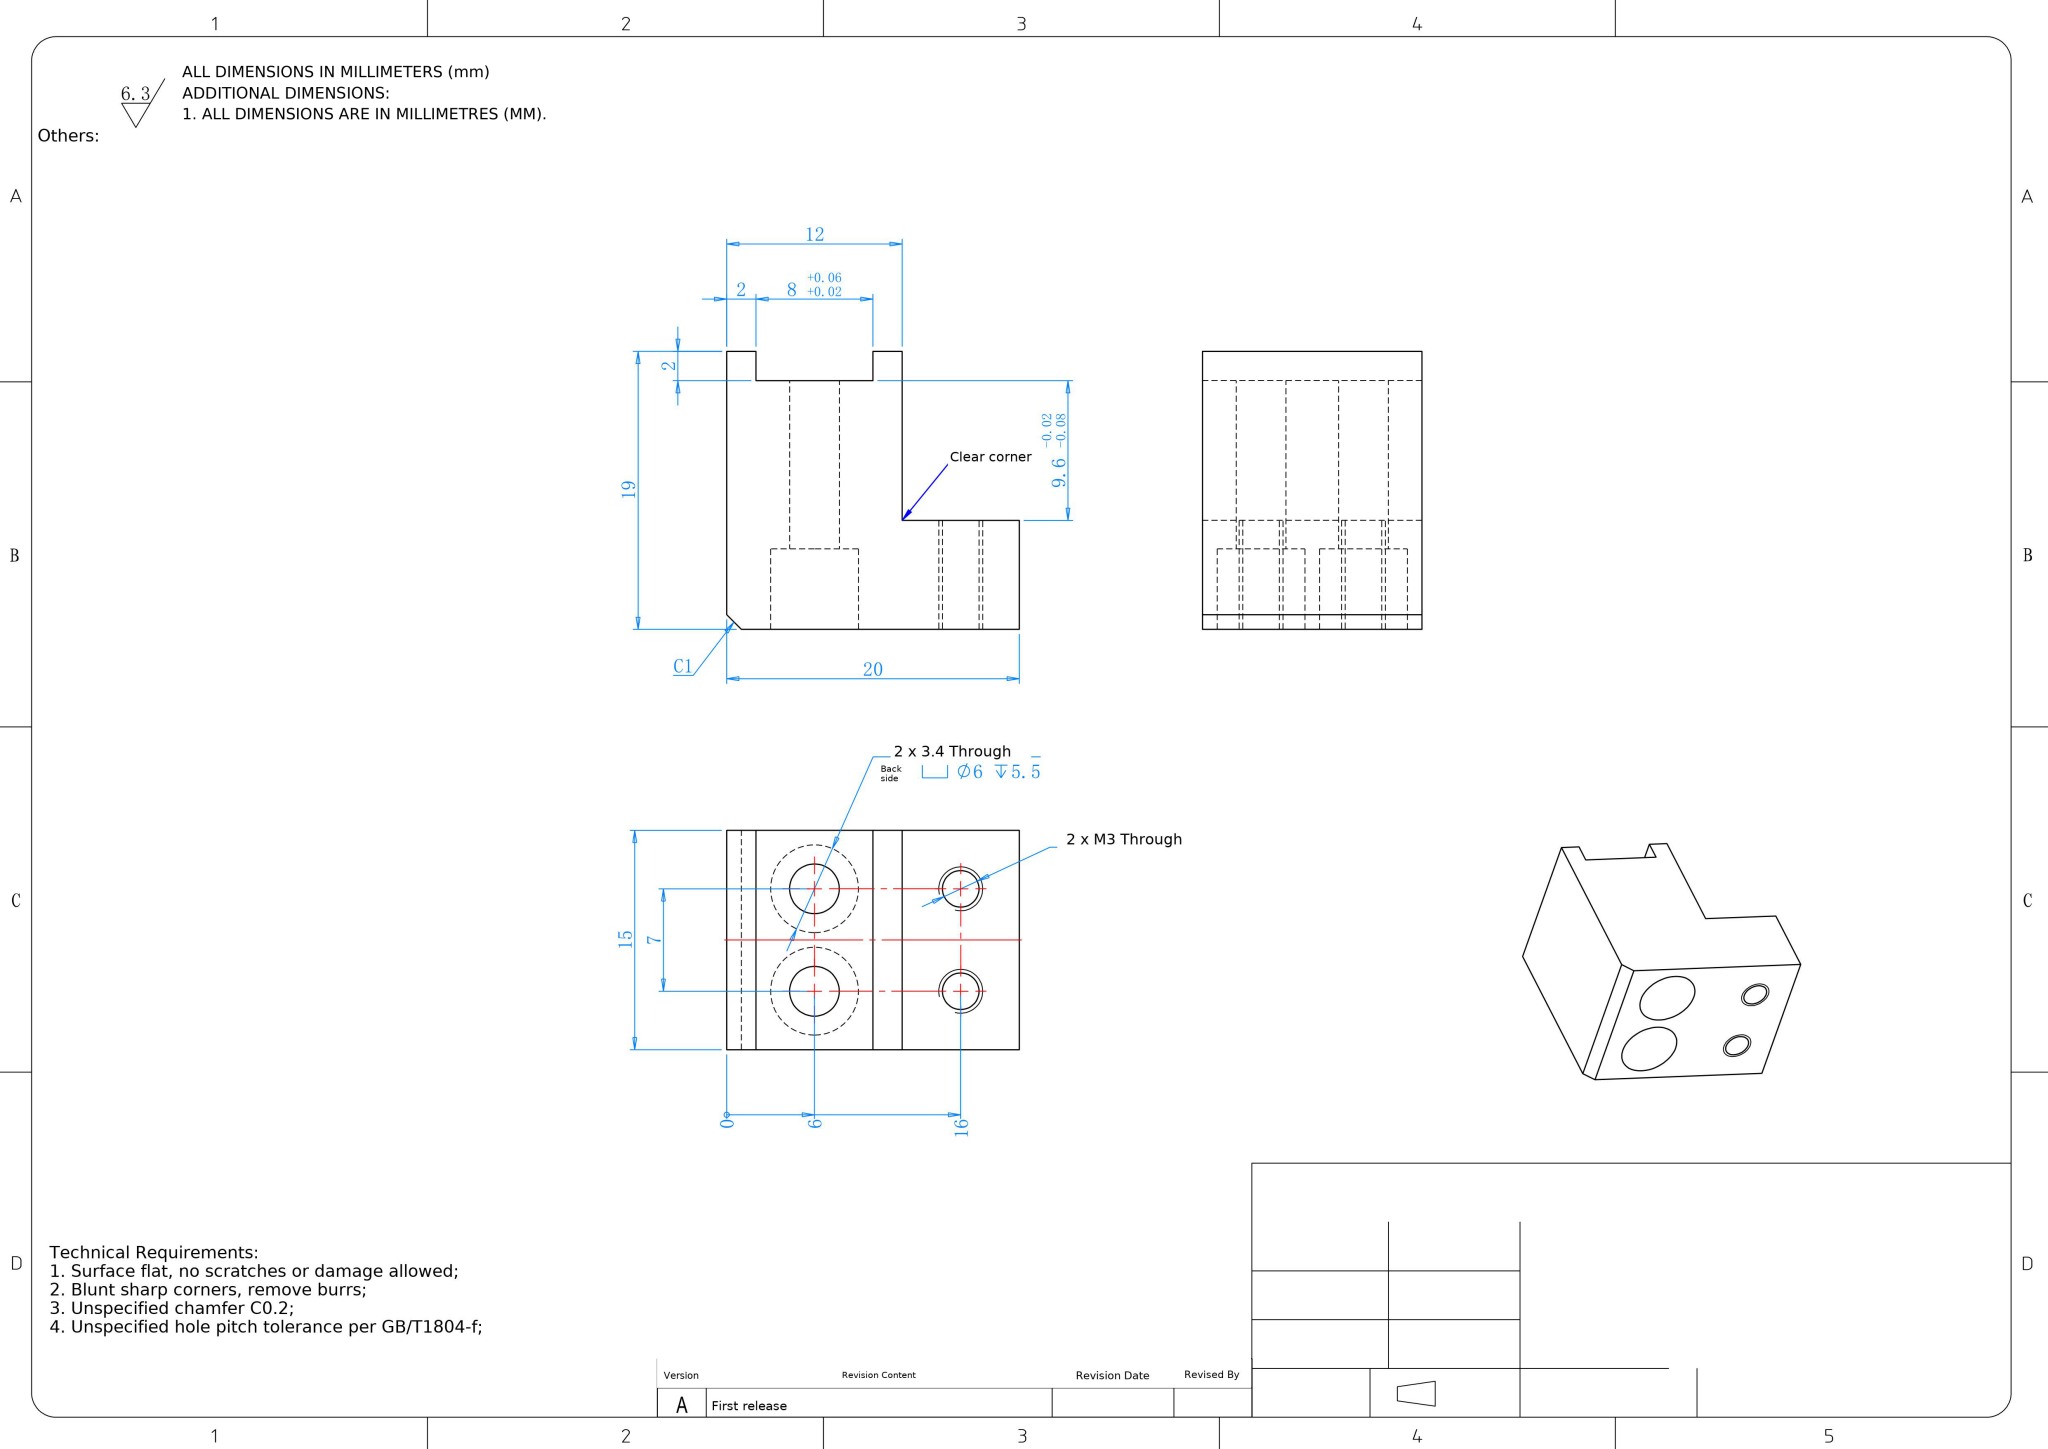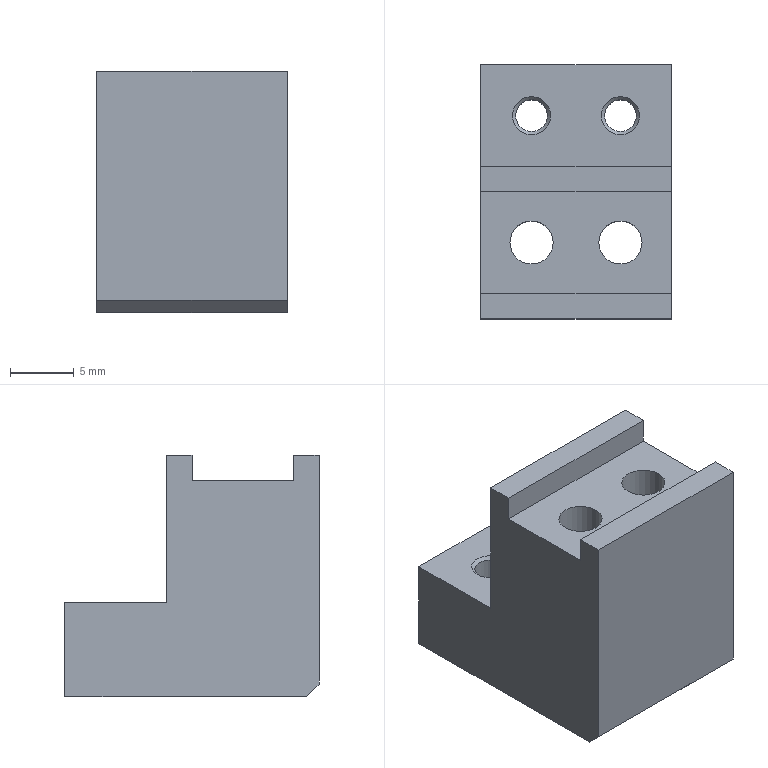Part | NX | mm | Stepped Dual-Tower Mounting Bracket | 1 solid | 25 faces | box 15 x 20 x 19 mm | volume 3467 mm3 | plane 15 | cylinder 6 | cone 4 | commonest cylinder face diameters 2.5 x2 3.4 x2 6 x2
STEP:
#1=CARTESIAN_POINT('',(0.,0.,0.));
#2=DIRECTION('',(0.,0.,1.));
#3=DIRECTION('',(1.,0.,0.));
#4=AXIS2_PLACEMENT_3D('',#1,#2,#3);
#5=(LENGTH_UNIT()NAMED_UNIT(*)SI_UNIT(.MILLI.,.METRE.));
#6=UNCERTAINTY_MEASURE_WITH_UNIT(LENGTH_MEASURE(0.00002),#5,'','');
#7=(NAMED_UNIT(*)PLANE_ANGLE_UNIT()SI_UNIT($,.RADIAN.));
#8=PLANE_ANGLE_MEASURE_WITH_UNIT(PLANE_ANGLE_MEASURE(0.01745),#7);
#9=DIMENSIONAL_EXPONENTS(0.,0.,0.,0.,0.,0.,0.);
#10=(CONVERSION_BASED_UNIT('',#8)NAMED_UNIT(#9)PLANE_ANGLE_UNIT());
#11=(NAMED_UNIT(*)SI_UNIT($,.STERADIAN.)SOLID_ANGLE_UNIT());
#12=(GEOMETRIC_REPRESENTATION_CONTEXT(3)GLOBAL_UNCERTAINTY_ASSIGNED_CONTEXT((#6))GLOBAL_UNIT_ASSIGNED_CONTEXT((#5,#10,#11))REPRESENTATION_CONTEXT('',''));
#13=SHAPE_REPRESENTATION('',(#4),#12);
#14=CARTESIAN_POINT('',(0.,-10.,19.));
#15=VERTEX_POINT('',#14);
#16=CARTESIAN_POINT('',(0.,-10.,1.));
#17=VERTEX_POINT('',#16);
#18=CARTESIAN_POINT('',(0.,-10.,19.));
#19=DIRECTION('',(0.,0.,-1.));
#20=VECTOR('',#19,1.);
#21=LINE('',#18,#20);
#22=EDGE_CURVE('',#15,#17,#21,.T.);
#23=ORIENTED_EDGE('',*,*,#22,.T.);
#24=CARTESIAN_POINT('',(15.,-10.,1.));
#25=VERTEX_POINT('',#24);
#26=CARTESIAN_POINT('',(15.,-10.,1.));
#27=DIRECTION('',(-1.,0.,0.));
#28=VECTOR('',#27,1.);
#29=LINE('',#26,#28);
#30=EDGE_CURVE('',#25,#17,#29,.T.);
#31=ORIENTED_EDGE('',*,*,#30,.F.);
#32=CARTESIAN_POINT('',(15.,-10.,19.));
#33=VERTEX_POINT('',#32);
#34=CARTESIAN_POINT('',(15.,-10.,19.));
#35=DIRECTION('',(0.,0.,-1.));
#36=VECTOR('',#35,1.);
#37=LINE('',#34,#36);
#38=EDGE_CURVE('',#33,#25,#37,.T.);
#39=ORIENTED_EDGE('',*,*,#38,.F.);
#40=CARTESIAN_POINT('',(15.,-10.,19.));
#41=DIRECTION('',(-1.,0.,0.));
#42=VECTOR('',#41,1.);
#43=LINE('',#40,#42);
#44=EDGE_CURVE('',#33,#15,#43,.T.);
#45=ORIENTED_EDGE('',*,*,#44,.T.);
#46=EDGE_LOOP('',(#23,#31,#39,#45));
#47=FACE_OUTER_BOUND('',#46,.T.);
#48=CARTESIAN_POINT('',(15.,-10.,19.));
#49=DIRECTION('',(0.,1.,0.));
#50=DIRECTION('',(0.,0.,1.));
#51=AXIS2_PLACEMENT_3D('',#48,#49,#50);
#52=PLANE('',#51);
#53=ADVANCED_FACE('',(#47),#52,.F.);
#54=CARTESIAN_POINT('',(0.,-9.,-0.));
#55=VERTEX_POINT('',#54);
#56=CARTESIAN_POINT('',(0.,-10.,1.));
#57=DIRECTION('',(0.,0.7071,-0.7071));
#58=VECTOR('',#57,1.);
#59=LINE('',#56,#58);
#60=EDGE_CURVE('',#17,#55,#59,.T.);
#61=ORIENTED_EDGE('',*,*,#60,.T.);
#62=CARTESIAN_POINT('',(15.,-9.,-0.));
#63=VERTEX_POINT('',#62);
#64=CARTESIAN_POINT('',(15.,-9.,-0.));
#65=DIRECTION('',(-1.,0.,0.));
#66=VECTOR('',#65,1.);
#67=LINE('',#64,#66);
#68=EDGE_CURVE('',#63,#55,#67,.T.);
#69=ORIENTED_EDGE('',*,*,#68,.F.);
#70=CARTESIAN_POINT('',(15.,-10.,1.));
#71=DIRECTION('',(0.,0.7071,-0.7071));
#72=VECTOR('',#71,1.);
#73=LINE('',#70,#72);
#74=EDGE_CURVE('',#25,#63,#73,.T.);
#75=ORIENTED_EDGE('',*,*,#74,.F.);
#76=ORIENTED_EDGE('',*,*,#30,.T.);
#77=EDGE_LOOP('',(#61,#69,#75,#76));
#78=FACE_OUTER_BOUND('',#77,.T.);
#79=CARTESIAN_POINT('',(15.,-10.,1.));
#80=DIRECTION('',(0.,0.7071,0.7071));
#81=DIRECTION('',(0.,-0.7071,0.7071));
#82=AXIS2_PLACEMENT_3D('',#79,#80,#81);
#83=PLANE('',#82);
#84=ADVANCED_FACE('',(#78),#83,.F.);
#85=CARTESIAN_POINT('',(7.,-4.,0.));
#86=VERTEX_POINT('',#85);
#87=CARTESIAN_POINT('',(4.,-4.,0.));
#88=DIRECTION('',(0.,0.,1.));
#89=DIRECTION('',(1.,0.,0.));
#90=AXIS2_PLACEMENT_3D('',#87,#88,#89);
#91=CIRCLE('',#90,3.);
#92=EDGE_CURVE('',#86,#86,#91,.T.);
#93=ORIENTED_EDGE('',*,*,#92,.T.);
#94=EDGE_LOOP('',(#93));
#95=FACE_BOUND('',#94,.T.);
#96=CARTESIAN_POINT('',(14.,-4.,0.));
#97=VERTEX_POINT('',#96);
#98=CARTESIAN_POINT('',(11.,-4.,0.));
#99=DIRECTION('',(0.,0.,1.));
#100=DIRECTION('',(1.,0.,0.));
#101=AXIS2_PLACEMENT_3D('',#98,#99,#100);
#102=CIRCLE('',#101,3.);
#103=EDGE_CURVE('',#97,#97,#102,.T.);
#104=ORIENTED_EDGE('',*,*,#103,.T.);
#105=EDGE_LOOP('',(#104));
#106=FACE_BOUND('',#105,.T.);
#107=CARTESIAN_POINT('',(5.5,6.,0.));
#108=VERTEX_POINT('',#107);
#109=CARTESIAN_POINT('',(4.,6.,0.));
#110=DIRECTION('',(0.,0.,1.));
#111=DIRECTION('',(1.,0.,0.));
#112=AXIS2_PLACEMENT_3D('',#109,#110,#111);
#113=CIRCLE('',#112,1.5);
#114=EDGE_CURVE('',#108,#108,#113,.T.);
#115=ORIENTED_EDGE('',*,*,#114,.T.);
#116=EDGE_LOOP('',(#115));
#117=FACE_BOUND('',#116,.T.);
#118=CARTESIAN_POINT('',(12.5,6.,0.));
#119=VERTEX_POINT('',#118);
#120=CARTESIAN_POINT('',(11.,6.,0.));
#121=DIRECTION('',(0.,0.,1.));
#122=DIRECTION('',(1.,0.,0.));
#123=AXIS2_PLACEMENT_3D('',#120,#121,#122);
#124=CIRCLE('',#123,1.5);
#125=EDGE_CURVE('',#119,#119,#124,.T.);
#126=ORIENTED_EDGE('',*,*,#125,.T.);
#127=EDGE_LOOP('',(#126));
#128=FACE_BOUND('',#127,.T.);
#129=CARTESIAN_POINT('',(0.,10.,0.));
#130=VERTEX_POINT('',#129);
#131=CARTESIAN_POINT('',(0.,-9.,0.));
#132=DIRECTION('',(0.,1.,0.));
#133=VECTOR('',#132,1.);
#134=LINE('',#131,#133);
#135=EDGE_CURVE('',#55,#130,#134,.T.);
#136=ORIENTED_EDGE('',*,*,#135,.T.);
#137=CARTESIAN_POINT('',(15.,10.,0.));
#138=VERTEX_POINT('',#137);
#139=CARTESIAN_POINT('',(15.,10.,0.));
#140=DIRECTION('',(-1.,0.,0.));
#141=VECTOR('',#140,1.);
#142=LINE('',#139,#141);
#143=EDGE_CURVE('',#138,#130,#142,.T.);
#144=ORIENTED_EDGE('',*,*,#143,.F.);
#145=CARTESIAN_POINT('',(15.,-9.,0.));
#146=DIRECTION('',(0.,1.,0.));
#147=VECTOR('',#146,1.);
#148=LINE('',#145,#147);
#149=EDGE_CURVE('',#63,#138,#148,.T.);
#150=ORIENTED_EDGE('',*,*,#149,.F.);
#151=ORIENTED_EDGE('',*,*,#68,.T.);
#152=EDGE_LOOP('',(#136,#144,#150,#151));
#153=FACE_BOUND('',#152,.T.);
#154=CARTESIAN_POINT('',(15.,-9.,0.));
#155=DIRECTION('',(0.,0.,1.));
#156=DIRECTION('',(1.,0.,0.));
#157=AXIS2_PLACEMENT_3D('',#154,#155,#156);
#158=PLANE('',#157);
#159=ADVANCED_FACE('',(#95,#106,#117,#128,#153),#158,.F.);
#160=CARTESIAN_POINT('',(0.,10.,7.4));
#161=VERTEX_POINT('',#160);
#162=CARTESIAN_POINT('',(0.,10.,0.));
#163=DIRECTION('',(0.,0.,1.));
#164=VECTOR('',#163,1.);
#165=LINE('',#162,#164);
#166=EDGE_CURVE('',#130,#161,#165,.T.);
#167=ORIENTED_EDGE('',*,*,#166,.T.);
#168=CARTESIAN_POINT('',(15.,10.,7.4));
#169=VERTEX_POINT('',#168);
#170=CARTESIAN_POINT('',(15.,10.,7.4));
#171=DIRECTION('',(-1.,0.,0.));
#172=VECTOR('',#171,1.);
#173=LINE('',#170,#172);
#174=EDGE_CURVE('',#169,#161,#173,.T.);
#175=ORIENTED_EDGE('',*,*,#174,.F.);
#176=CARTESIAN_POINT('',(15.,10.,0.));
#177=DIRECTION('',(0.,0.,1.));
#178=VECTOR('',#177,1.);
#179=LINE('',#176,#178);
#180=EDGE_CURVE('',#138,#169,#179,.T.);
#181=ORIENTED_EDGE('',*,*,#180,.F.);
#182=ORIENTED_EDGE('',*,*,#143,.T.);
#183=EDGE_LOOP('',(#167,#175,#181,#182));
#184=FACE_OUTER_BOUND('',#183,.T.);
#185=CARTESIAN_POINT('',(15.,10.,0.));
#186=DIRECTION('',(0.,-1.,0.));
#187=DIRECTION('',(0.,0.,-1.));
#188=AXIS2_PLACEMENT_3D('',#185,#186,#187);
#189=PLANE('',#188);
#190=ADVANCED_FACE('',(#184),#189,.F.);
#191=CARTESIAN_POINT('',(2.5,6.,7.4));
#192=VERTEX_POINT('',#191);
#193=CARTESIAN_POINT('',(4.,6.,7.4));
#194=DIRECTION('',(0.,0.,-1.));
#195=DIRECTION('',(-1.,0.,0.));
#196=AXIS2_PLACEMENT_3D('',#193,#194,#195);
#197=CIRCLE('',#196,1.5);
#198=EDGE_CURVE('',#192,#192,#197,.T.);
#199=ORIENTED_EDGE('',*,*,#198,.T.);
#200=EDGE_LOOP('',(#199));
#201=FACE_BOUND('',#200,.T.);
#202=CARTESIAN_POINT('',(9.5,6.,7.4));
#203=VERTEX_POINT('',#202);
#204=CARTESIAN_POINT('',(11.,6.,7.4));
#205=DIRECTION('',(0.,0.,-1.));
#206=DIRECTION('',(-1.,0.,0.));
#207=AXIS2_PLACEMENT_3D('',#204,#205,#206);
#208=CIRCLE('',#207,1.5);
#209=EDGE_CURVE('',#203,#203,#208,.T.);
#210=ORIENTED_EDGE('',*,*,#209,.T.);
#211=EDGE_LOOP('',(#210));
#212=FACE_BOUND('',#211,.T.);
#213=CARTESIAN_POINT('',(0.,2.,7.4));
#214=VERTEX_POINT('',#213);
#215=CARTESIAN_POINT('',(0.,10.,7.4));
#216=DIRECTION('',(0.,-1.,0.));
#217=VECTOR('',#216,1.);
#218=LINE('',#215,#217);
#219=EDGE_CURVE('',#161,#214,#218,.T.);
#220=ORIENTED_EDGE('',*,*,#219,.T.);
#221=CARTESIAN_POINT('',(15.,2.,7.4));
#222=VERTEX_POINT('',#221);
#223=CARTESIAN_POINT('',(15.,2.,7.4));
#224=DIRECTION('',(-1.,0.,0.));
#225=VECTOR('',#224,1.);
#226=LINE('',#223,#225);
#227=EDGE_CURVE('',#222,#214,#226,.T.);
#228=ORIENTED_EDGE('',*,*,#227,.F.);
#229=CARTESIAN_POINT('',(15.,10.,7.4));
#230=DIRECTION('',(0.,-1.,0.));
#231=VECTOR('',#230,1.);
#232=LINE('',#229,#231);
#233=EDGE_CURVE('',#169,#222,#232,.T.);
#234=ORIENTED_EDGE('',*,*,#233,.F.);
#235=ORIENTED_EDGE('',*,*,#174,.T.);
#236=EDGE_LOOP('',(#220,#228,#234,#235));
#237=FACE_BOUND('',#236,.T.);
#238=CARTESIAN_POINT('',(15.,10.,7.4));
#239=DIRECTION('',(0.,0.,-1.));
#240=DIRECTION('',(-1.,0.,0.));
#241=AXIS2_PLACEMENT_3D('',#238,#239,#240);
#242=PLANE('',#241);
#243=ADVANCED_FACE('',(#201,#212,#237),#242,.F.);
#244=CARTESIAN_POINT('',(0.,2.,19.));
#245=VERTEX_POINT('',#244);
#246=CARTESIAN_POINT('',(0.,2.,7.4));
#247=DIRECTION('',(0.,0.,1.));
#248=VECTOR('',#247,1.);
#249=LINE('',#246,#248);
#250=EDGE_CURVE('',#214,#245,#249,.T.);
#251=ORIENTED_EDGE('',*,*,#250,.T.);
#252=CARTESIAN_POINT('',(15.,2.,19.));
#253=VERTEX_POINT('',#252);
#254=CARTESIAN_POINT('',(15.,2.,19.));
#255=DIRECTION('',(-1.,0.,0.));
#256=VECTOR('',#255,1.);
#257=LINE('',#254,#256);
#258=EDGE_CURVE('',#253,#245,#257,.T.);
#259=ORIENTED_EDGE('',*,*,#258,.F.);
#260=CARTESIAN_POINT('',(15.,2.,7.4));
#261=DIRECTION('',(0.,0.,1.));
#262=VECTOR('',#261,1.);
#263=LINE('',#260,#262);
#264=EDGE_CURVE('',#222,#253,#263,.T.);
#265=ORIENTED_EDGE('',*,*,#264,.F.);
#266=ORIENTED_EDGE('',*,*,#227,.T.);
#267=EDGE_LOOP('',(#251,#259,#265,#266));
#268=FACE_OUTER_BOUND('',#267,.T.);
#269=CARTESIAN_POINT('',(15.,2.,7.4));
#270=DIRECTION('',(0.,-1.,0.));
#271=DIRECTION('',(0.,-0.,-1.));
#272=AXIS2_PLACEMENT_3D('',#269,#270,#271);
#273=PLANE('',#272);
#274=ADVANCED_FACE('',(#268),#273,.F.);
#275=CARTESIAN_POINT('',(0.,0.,19.));
#276=VERTEX_POINT('',#275);
#277=CARTESIAN_POINT('',(0.,2.,19.));
#278=DIRECTION('',(0.,-1.,0.));
#279=VECTOR('',#278,1.);
#280=LINE('',#277,#279);
#281=EDGE_CURVE('',#245,#276,#280,.T.);
#282=ORIENTED_EDGE('',*,*,#281,.T.);
#283=CARTESIAN_POINT('',(15.,0.,19.));
#284=VERTEX_POINT('',#283);
#285=CARTESIAN_POINT('',(15.,0.,19.));
#286=DIRECTION('',(-1.,0.,0.));
#287=VECTOR('',#286,1.);
#288=LINE('',#285,#287);
#289=EDGE_CURVE('',#284,#276,#288,.T.);
#290=ORIENTED_EDGE('',*,*,#289,.F.);
#291=CARTESIAN_POINT('',(15.,2.,19.));
#292=DIRECTION('',(0.,-1.,0.));
#293=VECTOR('',#292,1.);
#294=LINE('',#291,#293);
#295=EDGE_CURVE('',#253,#284,#294,.T.);
#296=ORIENTED_EDGE('',*,*,#295,.F.);
#297=ORIENTED_EDGE('',*,*,#258,.T.);
#298=EDGE_LOOP('',(#282,#290,#296,#297));
#299=FACE_OUTER_BOUND('',#298,.T.);
#300=CARTESIAN_POINT('',(15.,2.,19.));
#301=DIRECTION('',(0.,0.,-1.));
#302=DIRECTION('',(-1.,0.,0.));
#303=AXIS2_PLACEMENT_3D('',#300,#301,#302);
#304=PLANE('',#303);
#305=ADVANCED_FACE('',(#299),#304,.F.);
#306=CARTESIAN_POINT('',(0.,-0.,17.));
#307=VERTEX_POINT('',#306);
#308=CARTESIAN_POINT('',(0.,-0.,19.));
#309=DIRECTION('',(0.,0.,-1.));
#310=VECTOR('',#309,1.);
#311=LINE('',#308,#310);
#312=EDGE_CURVE('',#276,#307,#311,.T.);
#313=ORIENTED_EDGE('',*,*,#312,.T.);
#314=CARTESIAN_POINT('',(15.,-0.,17.));
#315=VERTEX_POINT('',#314);
#316=CARTESIAN_POINT('',(15.,-0.,17.));
#317=DIRECTION('',(-1.,0.,0.));
#318=VECTOR('',#317,1.);
#319=LINE('',#316,#318);
#320=EDGE_CURVE('',#315,#307,#319,.T.);
#321=ORIENTED_EDGE('',*,*,#320,.F.);
#322=CARTESIAN_POINT('',(15.,-0.,19.));
#323=DIRECTION('',(0.,0.,-1.));
#324=VECTOR('',#323,1.);
#325=LINE('',#322,#324);
#326=EDGE_CURVE('',#284,#315,#325,.T.);
#327=ORIENTED_EDGE('',*,*,#326,.F.);
#328=ORIENTED_EDGE('',*,*,#289,.T.);
#329=EDGE_LOOP('',(#313,#321,#327,#328));
#330=FACE_OUTER_BOUND('',#329,.T.);
#331=CARTESIAN_POINT('',(15.,-0.,19.));
#332=DIRECTION('',(0.,1.,0.));
#333=DIRECTION('',(0.,0.,1.));
#334=AXIS2_PLACEMENT_3D('',#331,#332,#333);
#335=PLANE('',#334);
#336=ADVANCED_FACE('',(#330),#335,.F.);
#337=CARTESIAN_POINT('',(2.3,-4.,17.));
#338=VERTEX_POINT('',#337);
#339=CARTESIAN_POINT('',(4.,-4.,17.));
#340=DIRECTION('',(0.,0.,-1.));
#341=DIRECTION('',(-1.,0.,0.));
#342=AXIS2_PLACEMENT_3D('',#339,#340,#341);
#343=CIRCLE('',#342,1.7);
#344=EDGE_CURVE('',#338,#338,#343,.T.);
#345=ORIENTED_EDGE('',*,*,#344,.T.);
#346=EDGE_LOOP('',(#345));
#347=FACE_BOUND('',#346,.T.);
#348=CARTESIAN_POINT('',(9.3,-4.,17.));
#349=VERTEX_POINT('',#348);
#350=CARTESIAN_POINT('',(11.,-4.,17.));
#351=DIRECTION('',(0.,0.,-1.));
#352=DIRECTION('',(-1.,0.,0.));
#353=AXIS2_PLACEMENT_3D('',#350,#351,#352);
#354=CIRCLE('',#353,1.7);
#355=EDGE_CURVE('',#349,#349,#354,.T.);
#356=ORIENTED_EDGE('',*,*,#355,.T.);
#357=EDGE_LOOP('',(#356));
#358=FACE_BOUND('',#357,.T.);
#359=CARTESIAN_POINT('',(0.,-8.,17.));
#360=VERTEX_POINT('',#359);
#361=CARTESIAN_POINT('',(0.,0.,17.));
#362=DIRECTION('',(0.,-1.,0.));
#363=VECTOR('',#362,1.);
#364=LINE('',#361,#363);
#365=EDGE_CURVE('',#307,#360,#364,.T.);
#366=ORIENTED_EDGE('',*,*,#365,.T.);
#367=CARTESIAN_POINT('',(15.,-8.,17.));
#368=VERTEX_POINT('',#367);
#369=CARTESIAN_POINT('',(15.,-8.,17.));
#370=DIRECTION('',(-1.,0.,0.));
#371=VECTOR('',#370,1.);
#372=LINE('',#369,#371);
#373=EDGE_CURVE('',#368,#360,#372,.T.);
#374=ORIENTED_EDGE('',*,*,#373,.F.);
#375=CARTESIAN_POINT('',(15.,0.,17.));
#376=DIRECTION('',(0.,-1.,0.));
#377=VECTOR('',#376,1.);
#378=LINE('',#375,#377);
#379=EDGE_CURVE('',#315,#368,#378,.T.);
#380=ORIENTED_EDGE('',*,*,#379,.F.);
#381=ORIENTED_EDGE('',*,*,#320,.T.);
#382=EDGE_LOOP('',(#366,#374,#380,#381));
#383=FACE_BOUND('',#382,.T.);
#384=CARTESIAN_POINT('',(15.,0.,17.));
#385=DIRECTION('',(0.,0.,-1.));
#386=DIRECTION('',(-1.,0.,0.));
#387=AXIS2_PLACEMENT_3D('',#384,#385,#386);
#388=PLANE('',#387);
#389=ADVANCED_FACE('',(#347,#358,#383),#388,.F.);
#390=CARTESIAN_POINT('',(0.,-8.,19.));
#391=VERTEX_POINT('',#390);
#392=CARTESIAN_POINT('',(0.,-8.,17.));
#393=DIRECTION('',(0.,0.,1.));
#394=VECTOR('',#393,1.);
#395=LINE('',#392,#394);
#396=EDGE_CURVE('',#360,#391,#395,.T.);
#397=ORIENTED_EDGE('',*,*,#396,.T.);
#398=CARTESIAN_POINT('',(15.,-8.,19.));
#399=VERTEX_POINT('',#398);
#400=CARTESIAN_POINT('',(15.,-8.,19.));
#401=DIRECTION('',(-1.,0.,0.));
#402=VECTOR('',#401,1.);
#403=LINE('',#400,#402);
#404=EDGE_CURVE('',#399,#391,#403,.T.);
#405=ORIENTED_EDGE('',*,*,#404,.F.);
#406=CARTESIAN_POINT('',(15.,-8.,17.));
#407=DIRECTION('',(0.,0.,1.));
#408=VECTOR('',#407,1.);
#409=LINE('',#406,#408);
#410=EDGE_CURVE('',#368,#399,#409,.T.);
#411=ORIENTED_EDGE('',*,*,#410,.F.);
#412=ORIENTED_EDGE('',*,*,#373,.T.);
#413=EDGE_LOOP('',(#397,#405,#411,#412));
#414=FACE_OUTER_BOUND('',#413,.T.);
#415=CARTESIAN_POINT('',(15.,-8.,17.));
#416=DIRECTION('',(0.,-1.,0.));
#417=DIRECTION('',(0.,0.,-1.));
#418=AXIS2_PLACEMENT_3D('',#415,#416,#417);
#419=PLANE('',#418);
#420=ADVANCED_FACE('',(#414),#419,.F.);
#421=CARTESIAN_POINT('',(0.,-8.,19.));
#422=DIRECTION('',(0.,-1.,0.));
#423=VECTOR('',#422,1.);
#424=LINE('',#421,#423);
#425=EDGE_CURVE('',#391,#15,#424,.T.);
#426=ORIENTED_EDGE('',*,*,#425,.T.);
#427=ORIENTED_EDGE('',*,*,#44,.F.);
#428=CARTESIAN_POINT('',(15.,-8.,19.));
#429=DIRECTION('',(0.,-1.,0.));
#430=VECTOR('',#429,1.);
#431=LINE('',#428,#430);
#432=EDGE_CURVE('',#399,#33,#431,.T.);
#433=ORIENTED_EDGE('',*,*,#432,.F.);
#434=ORIENTED_EDGE('',*,*,#404,.T.);
#435=EDGE_LOOP('',(#426,#427,#433,#434));
#436=FACE_OUTER_BOUND('',#435,.T.);
#437=CARTESIAN_POINT('',(15.,-8.,19.));
#438=DIRECTION('',(0.,0.,-1.));
#439=DIRECTION('',(-1.,0.,0.));
#440=AXIS2_PLACEMENT_3D('',#437,#438,#439);
#441=PLANE('',#440);
#442=ADVANCED_FACE('',(#436),#441,.F.);
#443=ORIENTED_EDGE('',*,*,#38,.T.);
#444=ORIENTED_EDGE('',*,*,#74,.T.);
#445=ORIENTED_EDGE('',*,*,#149,.T.);
#446=ORIENTED_EDGE('',*,*,#180,.T.);
#447=ORIENTED_EDGE('',*,*,#233,.T.);
#448=ORIENTED_EDGE('',*,*,#264,.T.);
#449=ORIENTED_EDGE('',*,*,#295,.T.);
#450=ORIENTED_EDGE('',*,*,#326,.T.);
#451=ORIENTED_EDGE('',*,*,#379,.T.);
#452=ORIENTED_EDGE('',*,*,#410,.T.);
#453=ORIENTED_EDGE('',*,*,#432,.T.);
#454=EDGE_LOOP('',(#443,#444,#445,#446,#447,#448,#449,#450,#451,#452,#453));
#455=FACE_OUTER_BOUND('',#454,.T.);
#456=CARTESIAN_POINT('',(15.,0.,0.));
#457=DIRECTION('',(1.,0.,0.));
#458=DIRECTION('',(0.,0.,-1.));
#459=AXIS2_PLACEMENT_3D('',#456,#457,#458);
#460=PLANE('',#459);
#461=ADVANCED_FACE('',(#455),#460,.T.);
#462=ORIENTED_EDGE('',*,*,#22,.F.);
#463=ORIENTED_EDGE('',*,*,#425,.F.);
#464=ORIENTED_EDGE('',*,*,#396,.F.);
#465=ORIENTED_EDGE('',*,*,#365,.F.);
#466=ORIENTED_EDGE('',*,*,#312,.F.);
#467=ORIENTED_EDGE('',*,*,#281,.F.);
#468=ORIENTED_EDGE('',*,*,#250,.F.);
#469=ORIENTED_EDGE('',*,*,#219,.F.);
#470=ORIENTED_EDGE('',*,*,#166,.F.);
#471=ORIENTED_EDGE('',*,*,#135,.F.);
#472=ORIENTED_EDGE('',*,*,#60,.F.);
#473=EDGE_LOOP('',(#462,#463,#464,#465,#466,#467,#468,#469,#470,#471,#472));
#474=FACE_OUTER_BOUND('',#473,.T.);
#475=CARTESIAN_POINT('',(0.,0.,0.));
#476=DIRECTION('',(1.,0.,0.));
#477=DIRECTION('',(0.,0.,-1.));
#478=AXIS2_PLACEMENT_3D('',#475,#476,#477);
#479=PLANE('',#478);
#480=ADVANCED_FACE('',(#474),#479,.F.);
#481=CARTESIAN_POINT('',(12.25,6.,7.15));
#482=VERTEX_POINT('',#481);
#483=CARTESIAN_POINT('',(11.,6.,7.15));
#484=DIRECTION('',(0.,0.,1.));
#485=DIRECTION('',(1.,0.,0.));
#486=AXIS2_PLACEMENT_3D('',#483,#484,#485);
#487=CIRCLE('',#486,1.25);
#488=EDGE_CURVE('',#482,#482,#487,.T.);
#489=ORIENTED_EDGE('',*,*,#488,.T.);
#490=EDGE_LOOP('',(#489));
#491=FACE_BOUND('',#490,.T.);
#492=CARTESIAN_POINT('',(9.75,6.,0.25));
#493=VERTEX_POINT('',#492);
#494=CARTESIAN_POINT('',(11.,6.,0.25));
#495=DIRECTION('',(0.,0.,-1.));
#496=DIRECTION('',(-1.,0.,0.));
#497=AXIS2_PLACEMENT_3D('',#494,#495,#496);
#498=CIRCLE('',#497,1.25);
#499=EDGE_CURVE('',#493,#493,#498,.T.);
#500=ORIENTED_EDGE('',*,*,#499,.T.);
#501=EDGE_LOOP('',(#500));
#502=FACE_BOUND('',#501,.T.);
#503=CARTESIAN_POINT('',(11.,6.,0.));
#504=DIRECTION('',(0.,0.,1.));
#505=DIRECTION('',(1.,0.,0.));
#506=AXIS2_PLACEMENT_3D('',#503,#504,#505);
#507=CYLINDRICAL_SURFACE('',#506,1.25);
#508=ADVANCED_FACE('',(#491,#502),#507,.F.);
#509=ORIENTED_EDGE('',*,*,#499,.F.);
#510=EDGE_LOOP('',(#509));
#511=FACE_BOUND('',#510,.T.);
#512=ORIENTED_EDGE('',*,*,#125,.F.);
#513=EDGE_LOOP('',(#512));
#514=FACE_BOUND('',#513,.T.);
#515=CARTESIAN_POINT('',(11.,6.,1.5));
#516=DIRECTION('',(0.,0.,-1.));
#517=DIRECTION('',(-1.,0.,0.));
#518=AXIS2_PLACEMENT_3D('',#515,#516,#517);
#519=CONICAL_SURFACE('',#518,0.,45.);
#520=ADVANCED_FACE('',(#511,#514),#519,.F.);
#521=ORIENTED_EDGE('',*,*,#488,.F.);
#522=EDGE_LOOP('',(#521));
#523=FACE_BOUND('',#522,.T.);
#524=ORIENTED_EDGE('',*,*,#209,.F.);
#525=EDGE_LOOP('',(#524));
#526=FACE_BOUND('',#525,.T.);
#527=CARTESIAN_POINT('',(11.,6.,5.9));
#528=DIRECTION('',(0.,0.,1.));
#529=DIRECTION('',(1.,0.,0.));
#530=AXIS2_PLACEMENT_3D('',#527,#528,#529);
#531=CONICAL_SURFACE('',#530,0.,45.);
#532=ADVANCED_FACE('',(#523,#526),#531,.F.);
#533=CARTESIAN_POINT('',(5.25,6.,7.15));
#534=VERTEX_POINT('',#533);
#535=CARTESIAN_POINT('',(4.,6.,7.15));
#536=DIRECTION('',(0.,0.,1.));
#537=DIRECTION('',(1.,0.,0.));
#538=AXIS2_PLACEMENT_3D('',#535,#536,#537);
#539=CIRCLE('',#538,1.25);
#540=EDGE_CURVE('',#534,#534,#539,.T.);
#541=ORIENTED_EDGE('',*,*,#540,.T.);
#542=EDGE_LOOP('',(#541));
#543=FACE_BOUND('',#542,.T.);
#544=CARTESIAN_POINT('',(2.75,6.,0.25));
#545=VERTEX_POINT('',#544);
#546=CARTESIAN_POINT('',(4.,6.,0.25));
#547=DIRECTION('',(0.,0.,-1.));
#548=DIRECTION('',(-1.,0.,0.));
#549=AXIS2_PLACEMENT_3D('',#546,#547,#548);
#550=CIRCLE('',#549,1.25);
#551=EDGE_CURVE('',#545,#545,#550,.T.);
#552=ORIENTED_EDGE('',*,*,#551,.T.);
#553=EDGE_LOOP('',(#552));
#554=FACE_BOUND('',#553,.T.);
#555=CARTESIAN_POINT('',(4.,6.,0.));
#556=DIRECTION('',(0.,0.,1.));
#557=DIRECTION('',(1.,0.,0.));
#558=AXIS2_PLACEMENT_3D('',#555,#556,#557);
#559=CYLINDRICAL_SURFACE('',#558,1.25);
#560=ADVANCED_FACE('',(#543,#554),#559,.F.);
#561=ORIENTED_EDGE('',*,*,#551,.F.);
#562=EDGE_LOOP('',(#561));
#563=FACE_BOUND('',#562,.T.);
#564=ORIENTED_EDGE('',*,*,#114,.F.);
#565=EDGE_LOOP('',(#564));
#566=FACE_BOUND('',#565,.T.);
#567=CARTESIAN_POINT('',(4.,6.,1.5));
#568=DIRECTION('',(0.,0.,-1.));
#569=DIRECTION('',(-1.,0.,0.));
#570=AXIS2_PLACEMENT_3D('',#567,#568,#569);
#571=CONICAL_SURFACE('',#570,0.,45.);
#572=ADVANCED_FACE('',(#563,#566),#571,.F.);
#573=ORIENTED_EDGE('',*,*,#540,.F.);
#574=EDGE_LOOP('',(#573));
#575=FACE_BOUND('',#574,.T.);
#576=ORIENTED_EDGE('',*,*,#198,.F.);
#577=EDGE_LOOP('',(#576));
#578=FACE_BOUND('',#577,.T.);
#579=CARTESIAN_POINT('',(4.,6.,5.9));
#580=DIRECTION('',(0.,0.,1.));
#581=DIRECTION('',(1.,0.,0.));
#582=AXIS2_PLACEMENT_3D('',#579,#580,#581);
#583=CONICAL_SURFACE('',#582,0.,45.);
#584=ADVANCED_FACE('',(#575,#578),#583,.F.);
#585=CARTESIAN_POINT('',(12.7,-4.,5.5));
#586=VERTEX_POINT('',#585);
#587=CARTESIAN_POINT('',(11.,-4.,5.5));
#588=DIRECTION('',(0.,0.,-1.));
#589=DIRECTION('',(1.,0.,0.));
#590=AXIS2_PLACEMENT_3D('',#587,#588,#589);
#591=CIRCLE('',#590,1.7);
#592=EDGE_CURVE('',#586,#586,#591,.T.);
#593=ORIENTED_EDGE('',*,*,#592,.T.);
#594=EDGE_LOOP('',(#593));
#595=FACE_BOUND('',#594,.T.);
#596=ORIENTED_EDGE('',*,*,#355,.F.);
#597=EDGE_LOOP('',(#596));
#598=FACE_BOUND('',#597,.T.);
#599=CARTESIAN_POINT('',(11.,-4.,50.));
#600=DIRECTION('',(0.,0.,1.));
#601=DIRECTION('',(1.,0.,0.));
#602=AXIS2_PLACEMENT_3D('',#599,#600,#601);
#603=CYLINDRICAL_SURFACE('',#602,1.7);
#604=ADVANCED_FACE('',(#595,#598),#603,.F.);
#605=ORIENTED_EDGE('',*,*,#592,.F.);
#606=EDGE_LOOP('',(#605));
#607=FACE_BOUND('',#606,.T.);
#608=CARTESIAN_POINT('',(14.,-4.,5.5));
#609=VERTEX_POINT('',#608);
#610=CARTESIAN_POINT('',(11.,-4.,5.5));
#611=DIRECTION('',(0.,0.,-1.));
#612=DIRECTION('',(1.,0.,0.));
#613=AXIS2_PLACEMENT_3D('',#610,#611,#612);
#614=CIRCLE('',#613,3.);
#615=EDGE_CURVE('',#609,#609,#614,.T.);
#616=ORIENTED_EDGE('',*,*,#615,.T.);
#617=EDGE_LOOP('',(#616));
#618=FACE_BOUND('',#617,.T.);
#619=CARTESIAN_POINT('',(11.,-4.,5.5));
#620=DIRECTION('',(0.,0.,1.));
#621=DIRECTION('',(1.,0.,0.));
#622=AXIS2_PLACEMENT_3D('',#619,#620,#621);
#623=PLANE('',#622);
#624=ADVANCED_FACE('',(#607,#618),#623,.F.);
#625=ORIENTED_EDGE('',*,*,#615,.F.);
#626=EDGE_LOOP('',(#625));
#627=FACE_BOUND('',#626,.T.);
#628=ORIENTED_EDGE('',*,*,#103,.F.);
#629=EDGE_LOOP('',(#628));
#630=FACE_BOUND('',#629,.T.);
#631=CARTESIAN_POINT('',(11.,-4.,0.));
#632=DIRECTION('',(0.,0.,1.));
#633=DIRECTION('',(1.,0.,0.));
#634=AXIS2_PLACEMENT_3D('',#631,#632,#633);
#635=CYLINDRICAL_SURFACE('',#634,3.);
#636=ADVANCED_FACE('',(#627,#630),#635,.F.);
#637=CARTESIAN_POINT('',(5.7,-4.,5.5));
#638=VERTEX_POINT('',#637);
#639=CARTESIAN_POINT('',(4.,-4.,5.5));
#640=DIRECTION('',(0.,0.,-1.));
#641=DIRECTION('',(1.,0.,0.));
#642=AXIS2_PLACEMENT_3D('',#639,#640,#641);
#643=CIRCLE('',#642,1.7);
#644=EDGE_CURVE('',#638,#638,#643,.T.);
#645=ORIENTED_EDGE('',*,*,#644,.T.);
#646=EDGE_LOOP('',(#645));
#647=FACE_BOUND('',#646,.T.);
#648=ORIENTED_EDGE('',*,*,#344,.F.);
#649=EDGE_LOOP('',(#648));
#650=FACE_BOUND('',#649,.T.);
#651=CARTESIAN_POINT('',(4.,-4.,50.));
#652=DIRECTION('',(0.,0.,1.));
#653=DIRECTION('',(1.,0.,0.));
#654=AXIS2_PLACEMENT_3D('',#651,#652,#653);
#655=CYLINDRICAL_SURFACE('',#654,1.7);
#656=ADVANCED_FACE('',(#647,#650),#655,.F.);
#657=ORIENTED_EDGE('',*,*,#644,.F.);
#658=EDGE_LOOP('',(#657));
#659=FACE_BOUND('',#658,.T.);
#660=CARTESIAN_POINT('',(7.,-4.,5.5));
#661=VERTEX_POINT('',#660);
#662=CARTESIAN_POINT('',(4.,-4.,5.5));
#663=DIRECTION('',(0.,0.,-1.));
#664=DIRECTION('',(1.,0.,0.));
#665=AXIS2_PLACEMENT_3D('',#662,#663,#664);
#666=CIRCLE('',#665,3.);
#667=EDGE_CURVE('',#661,#661,#666,.T.);
#668=ORIENTED_EDGE('',*,*,#667,.T.);
#669=EDGE_LOOP('',(#668));
#670=FACE_BOUND('',#669,.T.);
#671=CARTESIAN_POINT('',(4.,-4.,5.5));
#672=DIRECTION('',(0.,0.,1.));
#673=DIRECTION('',(1.,0.,0.));
#674=AXIS2_PLACEMENT_3D('',#671,#672,#673);
#675=PLANE('',#674);
#676=ADVANCED_FACE('',(#659,#670),#675,.F.);
#677=ORIENTED_EDGE('',*,*,#667,.F.);
#678=EDGE_LOOP('',(#677));
#679=FACE_BOUND('',#678,.T.);
#680=ORIENTED_EDGE('',*,*,#92,.F.);
#681=EDGE_LOOP('',(#680));
#682=FACE_BOUND('',#681,.T.);
#683=CARTESIAN_POINT('',(4.,-4.,0.));
#684=DIRECTION('',(0.,0.,1.));
#685=DIRECTION('',(1.,0.,0.));
#686=AXIS2_PLACEMENT_3D('',#683,#684,#685);
#687=CYLINDRICAL_SURFACE('',#686,3.);
#688=ADVANCED_FACE('',(#679,#682),#687,.F.);
#689=CLOSED_SHELL('',(#53,#84,#159,#190,#243,#274,#305,#336,#389,#420,#442,#461,#480,#508,#520,#532,#560,#572,#584,#604,#624,#636,#656,#676,#688));
#690=MANIFOLD_SOLID_BREP('',#689);
#691=ADVANCED_BREP_SHAPE_REPRESENTATION('',(#690),#12);
#692=SHAPE_REPRESENTATION_RELATIONSHIP('','',#13,#691);
#693=CARTESIAN_POINT('',(0.,10.,19.));
#694=CARTESIAN_POINT('',(0.,-10.,0.));
#695=GEOMETRIC_CURVE_SET('',(#693,#694));
#696=GEOMETRICALLY_BOUNDED_WIREFRAME_SHAPE_REPRESENTATION('',(#695),#12);
#697=SHAPE_REPRESENTATION_RELATIONSHIP('','',#13,#696);
#698=PRESENTATION_LAYER_ASSIGNMENT('','',(#693,#694,#690));
#699=DRAUGHTING_PRE_DEFINED_COLOUR('');
#700=POINT_STYLE('',MARKER_TYPE(.PLUS.),POSITIVE_LENGTH_MEASURE(3.),#699);
#701=PRESENTATION_STYLE_ASSIGNMENT((#700));
#702=STYLED_ITEM('',(#701),#693);
#703=POINT_STYLE('',MARKER_TYPE(.PLUS.),POSITIVE_LENGTH_MEASURE(3.),#699);
#704=PRESENTATION_STYLE_ASSIGNMENT((#703));
#705=STYLED_ITEM('',(#704),#694);
#706=COLOUR_RGB('',1.,0.6,0.);
#707=FILL_AREA_STYLE_COLOUR('',#706);
#708=FILL_AREA_STYLE('',(#707));
#709=SURFACE_STYLE_FILL_AREA(#708);
#710=SURFACE_SIDE_STYLE('',(#709));
#711=SURFACE_STYLE_USAGE(.BOTH.,#710);
#712=PRESENTATION_STYLE_ASSIGNMENT((#711));
#713=STYLED_ITEM('',(#712),#690);
#714=MECHANICAL_DESIGN_GEOMETRIC_PRESENTATION_REPRESENTATION('',(#702,#705,#713),#12);